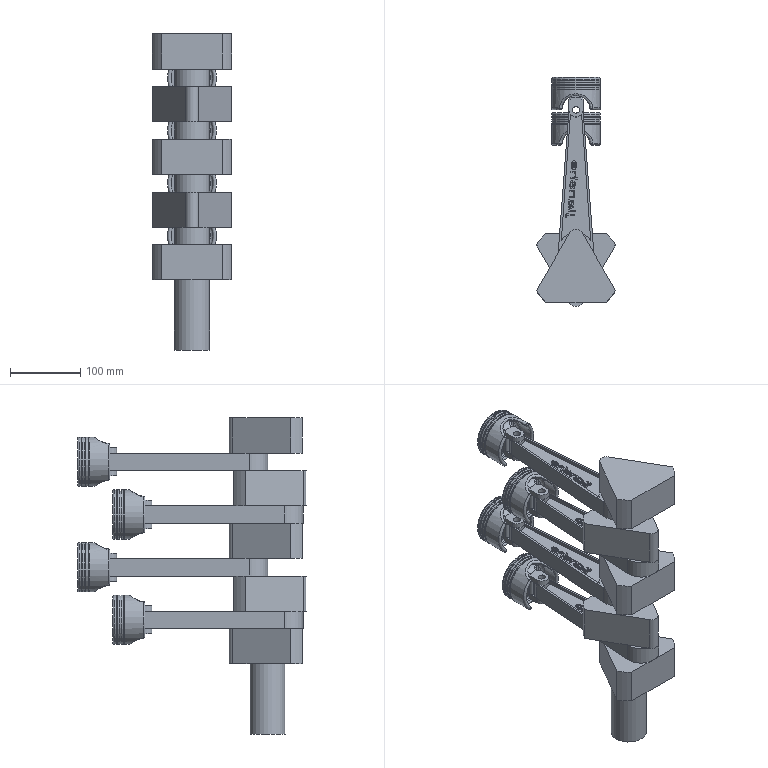Assembly | NX | mm | 9 component files | 18 solids | 975 faces | box 112.58 x 326 x 450 mm | volume 3028847 mm3 | plane 483 | other 264 | cylinder 124 | spline 72 | torus 16 | sphere 16 | commonest cylinder face diameters 20 x33 70 x16 10 x12 67.5 x12 130 x10 8 x8 30 x8 21 x8
Bill of materials:
unnamed part 1 | 4 |  | Hollow cylindrical cup-like body with a closed, rounded-edge end and an open end. Three shallow circumferential grooves run around the closed end. The open-end skirt has two opposed arched cutouts. Two parallel flat tabs with rounded ends and through-holes stick out past the open end from an internal rectangular boss. Overall the shape looks like a piston with a clevis-style pin lug.
unnamed part 2 | 1 |  | Stack of five flat, roughly triangular plates with rounded corners, spaced evenly along a central cylindrical shaft. Each plate is rotated 180 degrees from the one next to it. The shaft extends below the bottom plate as a plain round stub.
unnamed part 3 | 4 |  | Flat, tapered link or lever plate with rounded ends. The wide end has a large round through-hole and the narrow end a small one. A shallow pocket or recessed border runs along part of the top face, and raised lettering-like relief sits on the top face. The plate thickness is constant.
Mates:
1. concentric | p3 3 edge | p1 1 edge
2. concentric | p3 4 edge | p1 1 edge
3. concentric | p3 2 edge | p1 1 edge
4. concentric | p3 1 edge | p1 1 edge
5. concentric | p4 4 edge | p3 3 edge
6. concentric | p4 1 edge | p3 4 edge
7. concentric | p4 2 edge | p3 2 edge
8. concentric | p4 3 edge | p3 1 edge